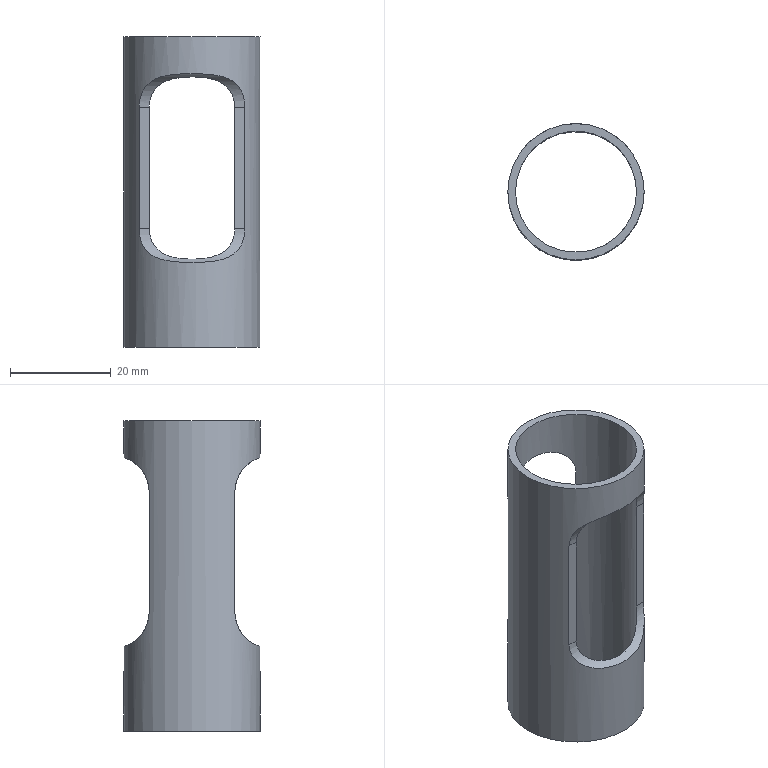Component | NX | LOWER_PISTON_CYLINDER_LINER | 1 solid | 12 faces | volume 5168 mm3 | cylinder 6 | plane 6 | commonest cylinder face diameters 14 x4 24 x1 27 x1